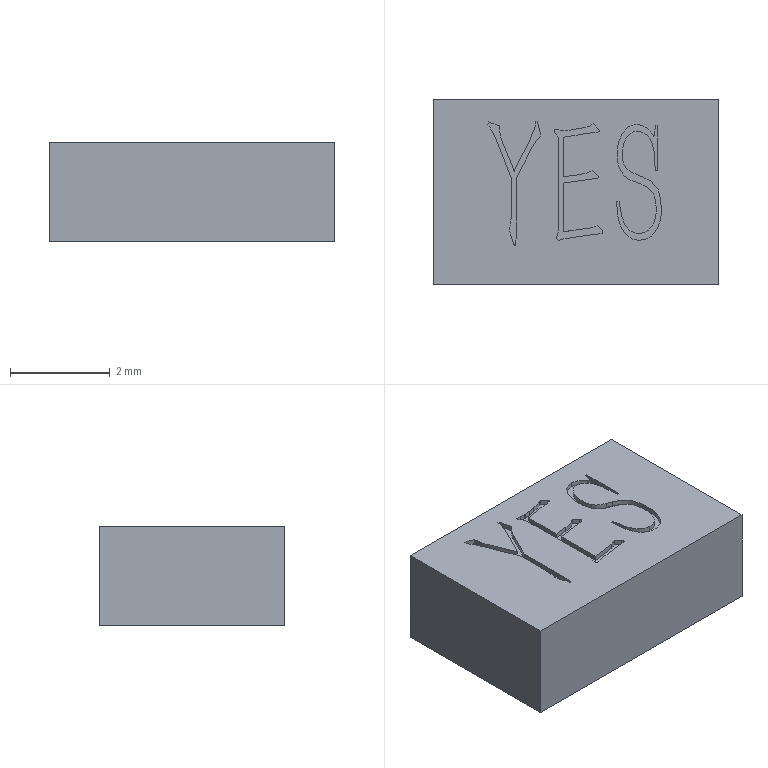Component | SolidWorks | Button2-1 | 1 solid | 89 faces | box 5.7 x 3.7 x 2 mm | volume 42 mm3 | plane 55 | spline 34
build123d program:
from build123d import *

# Parameters (mm, degrees)
SKETCH1_W           = 5.7
SKETCH1_H           = 3.7
BOSS_EXTRUDE1_DEPTH = 2
CUT_EXTRUDE1_DEPTH  = 0.1


with BuildPart() as part:
    # Sketch1 → Boss-Extrude1 (new body)
    with BuildSketch(Plane.XY):
        with Locations((2.85, 1.85)):
            Rectangle(SKETCH1_W, SKETCH1_H)
    extrude(amount=BOSS_EXTRUDE1_DEPTH)

    # Sketch2 → Cut-Extrude1 (cut)
    with BuildSketch(Plane.XY.offset(2)):
        with BuildLine():
            Line((1.655, 2.118), (1.658, 1.146))
            Line((1.658, 1.146), (1.651, 0.9093))
            add(Edge.make_bspline(
                [(1.651, 0.9093), (1.65, 0.8917), (1.648, 0.8597), (1.642, 0.8228), (1.637, 0.7994), (1.634, 0.7888), (1.628, 0.7815), (1.624, 0.7826), (1.622, 0.7831)],
                knots=[0, 0, 0, 0, 2.334, 4.235, 4.959, 5.465, 5.764, 6, 6, 6, 6], degree=3))
            add(Edge.make_bspline(
                [(1.622, 0.7831), (1.621, 0.7836), (1.617, 0.7849), (1.61, 0.7886), (1.604, 0.7989), (1.597, 0.8146), (1.592, 0.8406), (1.586, 0.8609), (1.583, 0.8731)],
                knots=[0, 0, 0, 0, 0.2675, 0.7025, 1.354, 2.279, 3.767, 6, 6, 6, 6], degree=3))
            Line((1.583, 0.8731), (1.54, 1.006))
            add(Edge.make_bspline(
                [(1.54, 1.006), (1.535, 1.019), (1.526, 1.042), (1.518, 1.072), (1.512, 1.094), (1.514, 1.106), (1.515, 1.111)],
                knots=[0, 0, 0, 0, 1.524, 2.689, 3.507, 4, 4, 4, 4], degree=3))
            Line((1.515, 1.111), (1.525, 1.146))
            add(Edge.make_bspline(
                [(1.525, 1.146), (1.527, 1.15), (1.53, 1.159), (1.533, 1.175), (1.536, 1.195), (1.538, 1.21), (1.54, 1.218)],
                knots=[0, 0, 0, 0, 0.6419, 1.535, 2.651, 4, 4, 4, 4], degree=3))
            Line((1.54, 1.218), (1.558, 1.358))
            add(Edge.make_bspline(
                [(1.558, 1.358), (1.558, 1.359), (1.558, 1.364), (1.558, 1.373), (1.558, 1.389), (1.558, 1.411), (1.558, 1.439), (1.558, 1.474), (1.558, 1.515), (1.558, 1.544), (1.558, 1.56)],
                knots=[0, 0, 0, 0, 0.127, 0.5079, 1.122, 2.011, 3.132, 4.508, 6.116, 8, 8, 8, 8], degree=3))
            Line((1.558, 1.56), (1.558, 2.11))
            Line((1.558, 2.11), (1.277, 2.837))
            add(Edge.make_bspline(
                [(1.277, 2.837), (1.271, 2.852), (1.259, 2.88), (1.243, 2.92), (1.228, 2.954), (1.211, 2.991), (1.19, 3.034), (1.163, 3.081), (1.14, 3.121), (1.125, 3.144), (1.119, 3.153)],
                knots=[0, 0, 0, 0, 1.116, 2.081, 2.921, 3.609, 4.867, 6.138, 7.243, 8, 8, 8, 8], degree=3))
            Line((1.119, 3.153), (1.087, 3.193))
            Line((1.087, 3.193), (1.101, 3.25))
            Line((1.101, 3.25), (1.313, 3.174))
            add(Edge.make_bspline(
                [(1.313, 3.174), (1.314, 3.16), (1.317, 3.134), (1.319, 3.103), (1.322, 3.078), (1.326, 3.056), (1.329, 3.03), (1.334, 2.99), (1.343, 2.939), (1.357, 2.901), (1.363, 2.883)],
                knots=[0, 0, 0, 0, 1.154, 2.091, 2.569, 3.164, 3.888, 4.729, 6.442, 8, 8, 8, 8], degree=3))
            Line((1.363, 2.883), (1.611, 2.268))
            Line((1.611, 2.268), (1.914, 2.862))
            add(Edge.make_bspline(
                [(1.914, 2.862), (1.918, 2.872), (1.928, 2.893), (1.944, 2.928), (1.962, 2.968), (1.982, 3.012), (2, 3.054), (2.014, 3.09), (2.024, 3.119), (2.027, 3.135), (2.029, 3.142)],
                knots=[0, 0, 0, 0, 0.8671, 1.872, 3.042, 4.362, 5.646, 6.673, 7.455, 8, 8, 8, 8], degree=3))
            Line((2.029, 3.142), (2.043, 3.257))
            Line((2.043, 3.257), (2.079, 3.257))
            Line((2.079, 3.257), (2.147, 2.969))
            add(Edge.make_bspline(
                [(2.147, 2.969), (2.138, 2.962), (2.121, 2.949), (2.1, 2.932), (2.083, 2.914), (2.068, 2.896), (2.05, 2.872), (2.023, 2.836), (1.992, 2.791), (1.973, 2.753), (1.964, 2.736)],
                knots=[0, 0, 0, 0, 0.9134, 1.741, 2.213, 2.829, 3.632, 4.588, 6.466, 8, 8, 8, 8], degree=3))
            Line((1.964, 2.736), (1.655, 2.118))
        make_face()
        with BuildLine():
            Line((2.603, 2.944), (2.603, 2.153))
            Line((2.603, 2.153), (2.905, 2.193))
            add(Edge.make_bspline(
                [(2.905, 2.193), (2.916, 2.194), (2.94, 2.198), (2.978, 2.205), (3.015, 2.214), (3.048, 2.223), (3.077, 2.233), (3.103, 2.243), (3.126, 2.254), (3.14, 2.264), (3.146, 2.268)],
                knots=[0, 0, 0, 0, 1.035, 2.296, 3.567, 4.627, 5.549, 6.429, 7.252, 8, 8, 8, 8], degree=3))
            Line((3.146, 2.268), (3.179, 2.286))
            Line((3.179, 2.286), (3.283, 2.182))
            add(Edge.make_bspline(
                [(3.283, 2.182), (3.288, 2.176), (3.296, 2.166), (3.3, 2.149), (3.297, 2.136), (3.289, 2.127), (3.278, 2.121), (3.27, 2.121), (3.265, 2.121)],
                knots=[0, 0, 0, 0, 1.598, 2.656, 3.463, 4.277, 5.07, 6, 6, 6, 6], degree=3))
            Line((3.265, 2.121), (2.603, 2.027))
            Line((2.603, 2.027), (2.603, 1.053))
            Line((2.603, 1.053), (3.139, 1.128))
            add(Edge.make_bspline(
                [(3.139, 1.128), (3.148, 1.13), (3.165, 1.133), (3.19, 1.141), (3.215, 1.152), (3.232, 1.16), (3.24, 1.164)],
                knots=[0, 0, 0, 0, 0.9523, 1.924, 2.936, 4, 4, 4, 4], degree=3))
            Line((3.24, 1.164), (3.272, 1.183))
            Line((3.272, 1.183), (3.373, 1.071))
            add(Edge.make_bspline(
                [(3.373, 1.071), (3.378, 1.065), (3.386, 1.055), (3.388, 1.038), (3.384, 1.027), (3.379, 1.017), (3.366, 1.014), (3.357, 1.013), (3.351, 1.013)],
                knots=[0, 0, 0, 0, 1.609, 2.656, 3.444, 4.084, 4.768, 6, 6, 6, 6], degree=3))
            Line((3.351, 1.013), (3.298, 1.01))
            add(Edge.make_bspline(
                [(3.298, 1.01), (3.282, 1.009), (3.25, 1.006), (3.198, 0.9998), (3.14, 0.9921), (3.075, 0.9838), (3.004, 0.9735), (2.926, 0.9619), (2.842, 0.9483), (2.784, 0.9391), (2.754, 0.9344)],
                knots=[0, 0, 0, 0, 0.6631, 1.429, 2.283, 3.238, 4.282, 5.428, 6.663, 8, 8, 8, 8], degree=3))
            Line((2.754, 0.9344), (2.589, 0.9056))
            add(Edge.make_bspline(
                [(2.589, 0.9056), (2.576, 0.9006), (2.553, 0.8917), (2.522, 0.8825), (2.495, 0.8838), (2.473, 0.8971), (2.463, 0.9244), (2.465, 0.9443), (2.466, 0.9557)],
                knots=[0, 0, 0, 0, 1.38, 2.456, 3.257, 4.014, 4.864, 6, 6, 6, 6], degree=3))
            add(Edge.make_bspline(
                [(2.466, 0.9557), (2.467, 0.9598), (2.469, 0.9715), (2.477, 0.9917), (2.484, 1.018), (2.491, 1.05), (2.495, 1.091), (2.498, 1.122), (2.499, 1.139)],
                knots=[0, 0, 0, 0, 0.3984, 1.132, 2.072, 3.033, 4.271, 6, 6, 6, 6], degree=3))
            Line((2.499, 1.139), (2.499, 1.208))
            add(Edge.make_bspline(
                [(2.499, 1.208), (2.5, 1.218), (2.501, 1.236), (2.501, 1.261), (2.503, 1.281), (2.503, 1.293), (2.503, 1.298)],
                knots=[0, 0, 0, 0, 1.326, 2.438, 3.314, 4, 4, 4, 4], degree=3))
            Line((2.503, 1.298), (2.499, 2.944))
            add(Edge.make_bspline(
                [(2.499, 2.944), (2.492, 2.953), (2.478, 2.97), (2.456, 2.993), (2.439, 3.016), (2.423, 3.034), (2.415, 3.052), (2.41, 3.068), (2.411, 3.082), (2.408, 3.096), (2.423, 3.106), (2.434, 3.104), (2.441, 3.102)],
                knots=[0, 0, 0, 0, 1.535, 3.086, 4.484, 5.549, 6.416, 7.188, 7.885, 8.433, 8.98, 10, 10, 10, 10], degree=3))
            Line((2.441, 3.102), (2.51, 3.092))
            add(Edge.make_bspline(
                [(2.51, 3.092), (2.525, 3.09), (2.551, 3.086), (2.586, 3.083), (2.612, 3.081), (2.626, 3.084), (2.632, 3.084)],
                knots=[0, 0, 0, 0, 1.483, 2.595, 3.408, 4, 4, 4, 4], degree=3))
            Line((2.632, 3.084), (2.643, 3.084))
            add(Edge.make_bspline(
                [(2.643, 3.084), (2.656, 3.085), (2.682, 3.085), (2.719, 3.085), (2.752, 3.089), (2.773, 3.093), (2.783, 3.096)],
                knots=[0, 0, 0, 0, 1.165, 2.193, 3.137, 4, 4, 4, 4], degree=3))
            Line((2.783, 3.096), (2.924, 3.121))
            add(Edge.make_bspline(
                [(2.924, 3.121), (2.937, 3.123), (2.962, 3.126), (2.996, 3.132), (3.028, 3.14), (3.06, 3.149), (3.093, 3.159), (3.122, 3.17), (3.145, 3.18), (3.159, 3.189), (3.164, 3.193)],
                knots=[0, 0, 0, 0, 1.33, 2.357, 3.309, 4.413, 5.543, 6.513, 7.35, 8, 8, 8, 8], degree=3))
            Line((3.164, 3.193), (3.197, 3.214))
            Line((3.197, 3.214), (3.301, 3.106))
            add(Edge.make_bspline(
                [(3.301, 3.106), (3.304, 3.1), (3.311, 3.09), (3.316, 3.075), (3.314, 3.063), (3.306, 3.055), (3.296, 3.049), (3.287, 3.049), (3.283, 3.049)],
                knots=[0, 0, 0, 0, 1.627, 2.653, 3.381, 4.196, 5.044, 6, 6, 6, 6], degree=3))
            Line((3.283, 3.049), (3.226, 3.041))
            add(Edge.make_bspline(
                [(3.226, 3.041), (3.213, 3.04), (3.19, 3.037), (3.157, 3.032), (3.129, 3.029), (3.106, 3.025), (3.087, 3.023), (3.073, 3.022), (3.063, 3.021), (3.058, 3.02), (3.056, 3.02)],
                knots=[0, 0, 0, 0, 1.762, 3.297, 4.631, 5.74, 6.619, 7.297, 7.749, 8, 8, 8, 8], degree=3))
            Line((3.056, 3.02), (2.603, 2.944))
        make_face()
        with BuildLine():
            Line((4.409, 2.959), (4.446, 3.178))
            Line((4.446, 3.178), (4.481, 3.174))
            Line((4.481, 3.174), (4.481, 2.276))
            Line((4.481, 2.276), (4.438, 2.272))
            Line((4.438, 2.272), (4.413, 2.653))
            add(Edge.make_bspline(
                [(4.413, 2.653), (4.41, 2.674), (4.404, 2.713), (4.392, 2.766), (4.381, 2.81), (4.363, 2.854), (4.338, 2.901), (4.3, 2.951), (4.255, 2.996), (4.202, 3.032), (4.144, 3.059), (4.103, 3.064), (4.082, 3.067)],
                knots=[0, 0, 0, 0, 1.116, 2.064, 2.832, 3.447, 4.519, 5.603, 6.709, 7.828, 8.938, 10, 10, 10, 10], degree=3))
            add(Edge.make_bspline(
                [(4.082, 3.067), (4.07, 3.066), (4.045, 3.065), (4.014, 3.058), (3.987, 3.048), (3.965, 3.036), (3.941, 3.019), (3.916, 2.998), (3.89, 2.974), (3.868, 2.947), (3.848, 2.916), (3.827, 2.873), (3.806, 2.817), (3.792, 2.759), (3.786, 2.711), (3.782, 2.67), (3.779, 2.625), (3.777, 2.575), (3.779, 2.524), (3.787, 2.475), (3.8, 2.427), (3.813, 2.398), (3.82, 2.383)],
                knots=[0, 0, 0, 0, 0.864, 1.774, 2.275, 2.882, 3.575, 4.376, 5.219, 6.056, 6.917, 7.795, 9.516, 11.157, 12.014, 12.981, 14.073, 15.277, 16.507, 17.699, 18.859, 20, 20, 20, 20], degree=3))
            add(Edge.make_bspline(
                [(3.82, 2.383), (3.827, 2.37), (3.842, 2.343), (3.869, 2.308), (3.901, 2.28), (3.946, 2.251), (4, 2.225), (4.042, 2.208), (4.061, 2.2)],
                knots=[0, 0, 0, 0, 0.8923, 1.74, 2.554, 3.354, 4.822, 6, 6, 6, 6], degree=3))
            Line((4.061, 2.2), (4.187, 2.149))
            add(Edge.make_bspline(
                [(4.187, 2.149), (4.202, 2.142), (4.232, 2.129), (4.274, 2.107), (4.312, 2.085), (4.356, 2.056), (4.404, 2.017), (4.452, 1.964), (4.491, 1.904), (4.515, 1.833), (4.534, 1.757), (4.547, 1.674), (4.556, 1.584), (4.559, 1.487), (4.558, 1.387), (4.545, 1.322), (4.539, 1.29)],
                knots=[0, 0, 0, 0, 0.7032, 1.354, 1.954, 2.507, 3.526, 4.489, 5.438, 6.454, 7.532, 8.673, 9.9, 11.268, 12.658, 14, 14, 14, 14], degree=3))
            add(Edge.make_bspline(
                [(4.539, 1.29), (4.531, 1.258), (4.516, 1.196), (4.483, 1.124), (4.454, 1.074), (4.433, 1.041), (4.411, 1.013), (4.383, 0.9799), (4.34, 0.945), (4.29, 0.9173), (4.244, 0.9001), (4.206, 0.8902), (4.165, 0.8852), (4.136, 0.8843), (4.122, 0.8838)],
                knots=[0, 0, 0, 0, 1.868, 3.619, 4.43, 5.163, 5.83, 6.429, 7.607, 8.939, 9.658, 10.394, 11.175, 12, 12, 12, 12], degree=3))
            add(Edge.make_bspline(
                [(4.122, 0.8838), (4.105, 0.8839), (4.073, 0.8841), (4.026, 0.8916), (3.982, 0.9055), (3.941, 0.9261), (3.902, 0.9519), (3.867, 0.9825), (3.834, 1.018), (3.802, 1.056), (3.775, 1.1), (3.75, 1.148), (3.729, 1.2), (3.705, 1.273), (3.685, 1.366), (3.679, 1.441), (3.676, 1.477)],
                knots=[0, 0, 0, 0, 0.8339, 1.632, 2.411, 3.189, 3.973, 4.77, 5.584, 6.428, 7.308, 8.216, 9.166, 10.157, 12.133, 14, 14, 14, 14], degree=3))
            Line((3.676, 1.477), (3.661, 1.668))
            Line((3.661, 1.668), (3.712, 1.668))
            add(Edge.make_bspline(
                [(3.712, 1.668), (3.715, 1.645), (3.72, 1.602), (3.73, 1.539), (3.74, 1.482), (3.752, 1.413), (3.771, 1.335), (3.801, 1.25), (3.84, 1.176), (3.881, 1.123), (3.917, 1.087), (3.946, 1.066), (3.974, 1.048), (4.011, 1.033), (4.059, 1.02), (4.096, 1.021), (4.115, 1.021)],
                knots=[0, 0, 0, 0, 1.135, 2.183, 3.161, 4.052, 5.676, 7.155, 8.522, 9.84, 10.472, 11.06, 11.601, 12.121, 13.087, 14, 14, 14, 14], degree=3))
            add(Edge.make_bspline(
                [(4.115, 1.021), (4.131, 1.021), (4.162, 1.022), (4.206, 1.032), (4.247, 1.046), (4.283, 1.068), (4.315, 1.095), (4.344, 1.127), (4.37, 1.162), (4.392, 1.202), (4.412, 1.243), (4.428, 1.283), (4.44, 1.323), (4.448, 1.362), (4.453, 1.403), (4.456, 1.446), (4.458, 1.493), (4.457, 1.525), (4.456, 1.542)],
                knots=[0, 0, 0, 0, 1.108, 2.126, 3.098, 4.036, 4.985, 5.948, 6.947, 7.997, 9.046, 10.05, 10.988, 11.882, 12.789, 13.788, 14.845, 16, 16, 16, 16], degree=3))
            add(Edge.make_bspline(
                [(4.456, 1.542), (4.454, 1.569), (4.451, 1.618), (4.44, 1.685), (4.426, 1.742), (4.407, 1.789), (4.385, 1.827), (4.362, 1.862), (4.335, 1.893), (4.305, 1.92), (4.272, 1.945), (4.235, 1.968), (4.193, 1.99), (4.163, 2.003), (4.147, 2.009)],
                knots=[0, 0, 0, 0, 1.578, 2.946, 4.098, 5.071, 5.936, 6.762, 7.575, 8.365, 9.177, 10.055, 10.991, 12, 12, 12, 12], degree=3))
            Line((4.147, 2.009), (3.992, 2.067))
            add(Edge.make_bspline(
                [(3.992, 2.067), (3.968, 2.077), (3.92, 2.098), (3.855, 2.141), (3.798, 2.192), (3.752, 2.254), (3.717, 2.326), (3.696, 2.394), (3.684, 2.455), (3.678, 2.507), (3.675, 2.564), (3.675, 2.603), (3.676, 2.624)],
                knots=[0, 0, 0, 0, 1.142, 2.262, 3.359, 4.445, 5.59, 6.836, 7.519, 8.279, 9.098, 10, 10, 10, 10], degree=3))
            add(Edge.make_bspline(
                [(3.676, 2.624), (3.676, 2.642), (3.676, 2.677), (3.68, 2.727), (3.686, 2.773), (3.698, 2.83), (3.718, 2.896), (3.749, 2.97), (3.786, 3.036), (3.828, 3.092), (3.876, 3.135), (3.92, 3.166), (3.96, 3.183), (3.994, 3.193), (4.031, 3.198), (4.058, 3.199), (4.072, 3.199)],
                knots=[0, 0, 0, 0, 0.9712, 1.877, 2.722, 3.497, 4.993, 6.466, 7.856, 9.083, 10.219, 11.35, 11.94, 12.569, 13.259, 14, 14, 14, 14], degree=3))
            add(Edge.make_bspline(
                [(4.072, 3.199), (4.087, 3.198), (4.117, 3.194), (4.162, 3.182), (4.205, 3.165), (4.246, 3.141), (4.283, 3.115), (4.316, 3.087), (4.344, 3.058), (4.359, 3.037), (4.366, 3.027)],
                knots=[0, 0, 0, 0, 1.05, 2.088, 3.146, 4.218, 5.268, 6.247, 7.154, 8, 8, 8, 8], degree=3))
            Line((4.366, 3.027), (4.409, 2.959))
        make_face()
    extrude(amount=-CUT_EXTRUDE1_DEPTH, mode=Mode.SUBTRACT)


solid = part.part

# Placed as in the assembly
solid = solid.moved(Location((-81.206, -4.714, 277.152), (0, 0, 0)))